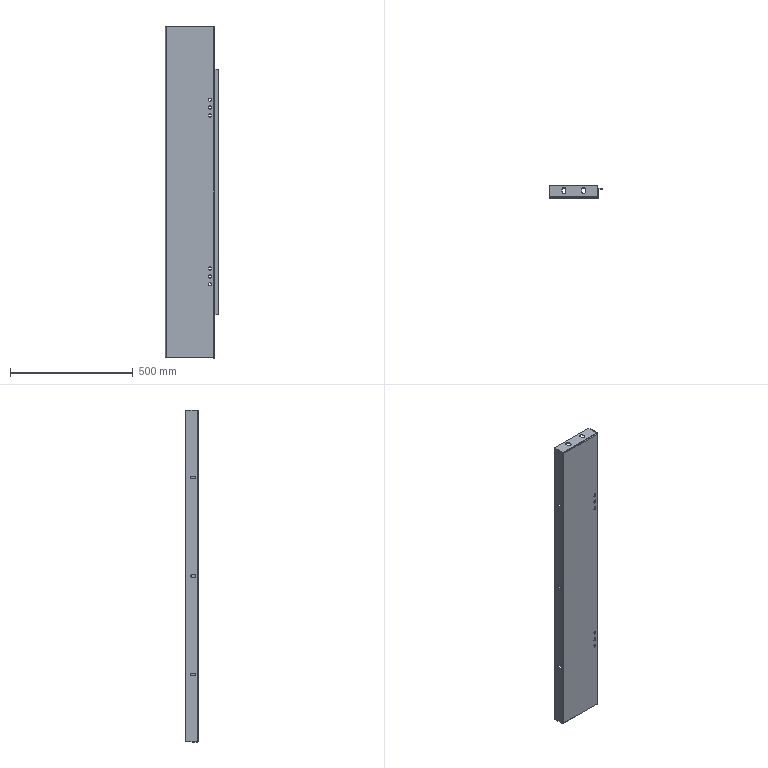Component | SolidWorks | HingeColumn-1 | 1 solid | 136 faces | volume 828754 mm3 | plane 74 | cylinder 58 | spline 4 | commonest cylinder face diameters 10 x18 9 x18 16 x12 4 x5 8 x5 | material Plain Carbon Steel